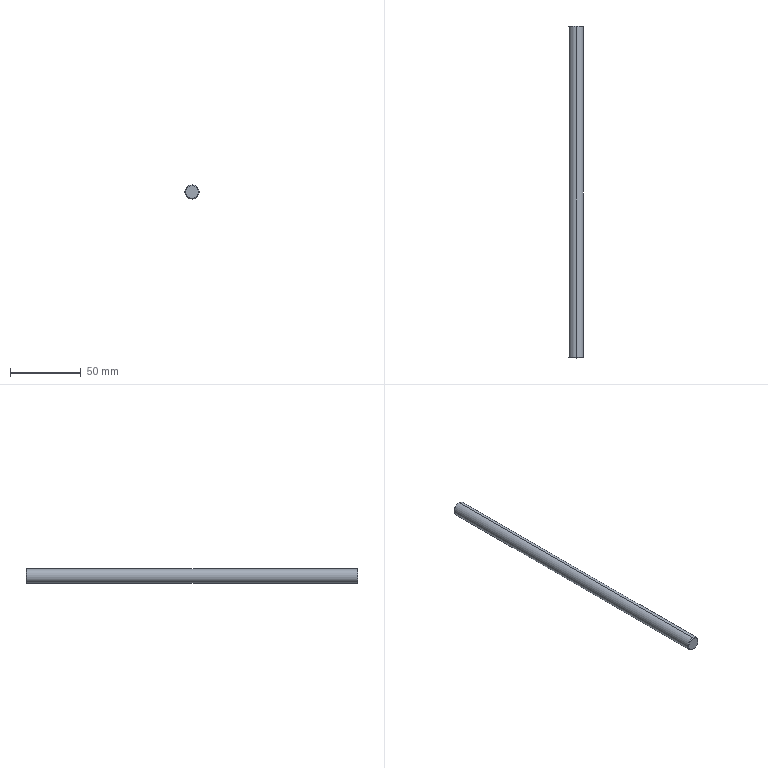Component | SolidWorks | STB-08-020-2 | 1 solid | 8 faces | box 10 x 235 x 10 mm | volume 18449 mm3 | cone 4 | cylinder 2 | plane 2 | commonest cylinder face diameters 10 x2
build123d program:
from build123d import *

# Parameters (mm, degrees)
SKETCH1_R           = 5
BOSS_EXTRUDE1_DEPTH = 117.5
CHAMFER1_SIZE       = 0.5


with BuildPart() as part:
    # Sketch1 → Boss-Extrude1 (new, symmetric)
    with BuildSketch(Plane(origin=(0, 0, 0), x_dir=(1, 0, 0), z_dir=(0, 1, 0))):
        with Locations(Location((0, 0, 0), (0, 0, 90))):
            Circle(SKETCH1_R)
    extrude(amount=BOSS_EXTRUDE1_DEPTH, both=True)

    # Chamfer1
    chamfer1_edges = [part.edges().sort_by_distance(p)[0] for p in [
        (0, -117.5, 5),
        (0, 117.5, 5),
    ]]
    chamfer(chamfer1_edges, length=CHAMFER1_SIZE)


solid = part.part

# Placed as in the assembly
solid = solid.moved(Location((-59.904, 349.499, -12), (0, 0, 0)))
STEP:
#1=COLOUR_RGB('',0.7922,0.8196,0.9333);
#2=FILL_AREA_STYLE_COLOUR('',#1);
#3=FILL_AREA_STYLE('',(#2));
#4=SURFACE_STYLE_FILL_AREA(#3);
#5=SURFACE_SIDE_STYLE('',(#4));
#6=SURFACE_STYLE_USAGE(.BOTH.,#5);
#7=PRESENTATION_STYLE_ASSIGNMENT((#6));
#8=CARTESIAN_POINT('',(-2.358,18.386,-0.2953));
#9=VERTEX_POINT('',#8);
#10=CARTESIAN_POINT('',(-2.358,18.386,-0.6496));
#11=VERTEX_POINT('',#10);
#12=CARTESIAN_POINT('',(-2.358,18.386,-0.4724));
#13=DIRECTION('',(0.,1.,0.));
#14=DIRECTION('',(0.,0.,1.));
#15=AXIS2_PLACEMENT_3D('',#12,#13,#14);
#16=CIRCLE('',#15,0.1772);
#17=EDGE_CURVE('',#9,#11,#16,.T.);
#18=ORIENTED_EDGE('',*,*,#17,.F.);
#19=CARTESIAN_POINT('',(-2.358,18.366,-0.2756));
#20=VERTEX_POINT('',#19);
#21=CARTESIAN_POINT('',(-2.358,18.386,-0.2953));
#22=DIRECTION('',(0.,-0.7071,0.7071));
#23=VECTOR('',#22,39.37);
#24=LINE('',#21,#23);
#25=EDGE_CURVE('',#9,#20,#24,.T.);
#26=ORIENTED_EDGE('',*,*,#25,.T.);
#27=CARTESIAN_POINT('',(-2.358,18.366,-0.6693));
#28=VERTEX_POINT('',#27);
#29=CARTESIAN_POINT('',(-2.358,18.366,-0.4724));
#30=DIRECTION('',(0.,-1.,0.));
#31=DIRECTION('',(0.,0.,1.));
#32=AXIS2_PLACEMENT_3D('',#29,#30,#31);
#33=CIRCLE('',#32,0.1969);
#34=EDGE_CURVE('',#28,#20,#33,.T.);
#35=ORIENTED_EDGE('',*,*,#34,.F.);
#36=CARTESIAN_POINT('',(-2.358,18.386,-0.6496));
#37=DIRECTION('',(0.,-0.7071,-0.7071));
#38=VECTOR('',#37,39.37);
#39=LINE('',#36,#38);
#40=EDGE_CURVE('',#11,#28,#39,.T.);
#41=ORIENTED_EDGE('',*,*,#40,.F.);
#42=EDGE_LOOP('',(#18,#26,#35,#41));
#43=FACE_OUTER_BOUND('',#42,.T.);
#44=CARTESIAN_POINT('',(-2.358,18.386,-0.4724));
#45=DIRECTION('',(0.,-1.,0.));
#46=DIRECTION('',(0.,0.,-1.));
#47=AXIS2_PLACEMENT_3D('',#44,#45,#46);
#48=CONICAL_SURFACE('',#47,0.1772,0.7854);
#49=ADVANCED_FACE('',(#43),#48,.T.);
#50=CARTESIAN_POINT('',(-2.358,9.134,-0.6496));
#51=VERTEX_POINT('',#50);
#52=CARTESIAN_POINT('',(-2.358,9.134,-0.2953));
#53=VERTEX_POINT('',#52);
#54=CARTESIAN_POINT('',(-2.358,9.134,-0.4724));
#55=DIRECTION('',(0.,-1.,0.));
#56=DIRECTION('',(0.,0.,1.));
#57=AXIS2_PLACEMENT_3D('',#54,#55,#56);
#58=CIRCLE('',#57,0.1772);
#59=EDGE_CURVE('',#51,#53,#58,.T.);
#60=ORIENTED_EDGE('',*,*,#59,.F.);
#61=CARTESIAN_POINT('',(-2.358,9.153,-0.6693));
#62=VERTEX_POINT('',#61);
#63=CARTESIAN_POINT('',(-2.358,9.153,-0.6693));
#64=DIRECTION('',(0.,0.7071,-0.7071));
#65=VECTOR('',#64,39.37);
#66=LINE('',#63,#65);
#67=EDGE_CURVE('',#51,#62,#66,.T.);
#68=ORIENTED_EDGE('',*,*,#67,.T.);
#69=CARTESIAN_POINT('',(-2.358,9.153,-0.2756));
#70=VERTEX_POINT('',#69);
#71=CARTESIAN_POINT('',(-2.358,9.153,-0.4724));
#72=DIRECTION('',(0.,1.,0.));
#73=DIRECTION('',(0.,0.,1.));
#74=AXIS2_PLACEMENT_3D('',#71,#72,#73);
#75=CIRCLE('',#74,0.1969);
#76=EDGE_CURVE('',#70,#62,#75,.T.);
#77=ORIENTED_EDGE('',*,*,#76,.F.);
#78=CARTESIAN_POINT('',(-2.358,9.153,-0.2756));
#79=DIRECTION('',(0.,0.7071,0.7071));
#80=VECTOR('',#79,39.37);
#81=LINE('',#78,#80);
#82=EDGE_CURVE('',#53,#70,#81,.T.);
#83=ORIENTED_EDGE('',*,*,#82,.F.);
#84=EDGE_LOOP('',(#60,#68,#77,#83));
#85=FACE_OUTER_BOUND('',#84,.T.);
#86=CARTESIAN_POINT('',(-2.358,9.153,-0.4724));
#87=DIRECTION('',(0.,1.,0.));
#88=DIRECTION('',(0.,0.,1.));
#89=AXIS2_PLACEMENT_3D('',#86,#87,#88);
#90=CONICAL_SURFACE('',#89,0.1969,0.7854);
#91=ADVANCED_FACE('',(#85),#90,.T.);
#92=ORIENTED_EDGE('',*,*,#34,.T.);
#93=CARTESIAN_POINT('',(-2.358,18.386,-0.2756));
#94=DIRECTION('',(0.,-1.,0.));
#95=VECTOR('',#94,39.37);
#96=LINE('',#93,#95);
#97=EDGE_CURVE('',#20,#70,#96,.T.);
#98=ORIENTED_EDGE('',*,*,#97,.T.);
#99=ORIENTED_EDGE('',*,*,#76,.T.);
#100=CARTESIAN_POINT('',(-2.358,18.386,-0.6693));
#101=DIRECTION('',(0.,-1.,0.));
#102=VECTOR('',#101,39.37);
#103=LINE('',#100,#102);
#104=EDGE_CURVE('',#28,#62,#103,.T.);
#105=ORIENTED_EDGE('',*,*,#104,.F.);
#106=EDGE_LOOP('',(#92,#98,#99,#105));
#107=FACE_OUTER_BOUND('',#106,.T.);
#108=CARTESIAN_POINT('',(-2.358,18.386,-0.4724));
#109=DIRECTION('',(0.,-1.,0.));
#110=DIRECTION('',(0.,0.,-1.));
#111=AXIS2_PLACEMENT_3D('',#108,#109,#110);
#112=CYLINDRICAL_SURFACE('',#111,0.1969);
#113=ADVANCED_FACE('',(#107),#112,.T.);
#114=ORIENTED_EDGE('',*,*,#97,.F.);
#115=CARTESIAN_POINT('',(-2.358,18.366,-0.4724));
#116=DIRECTION('',(0.,-1.,0.));
#117=DIRECTION('',(0.,0.,1.));
#118=AXIS2_PLACEMENT_3D('',#115,#116,#117);
#119=CIRCLE('',#118,0.1969);
#120=EDGE_CURVE('',#20,#28,#119,.T.);
#121=ORIENTED_EDGE('',*,*,#120,.T.);
#122=ORIENTED_EDGE('',*,*,#104,.T.);
#123=CARTESIAN_POINT('',(-2.358,9.153,-0.4724));
#124=DIRECTION('',(0.,1.,0.));
#125=DIRECTION('',(0.,0.,1.));
#126=AXIS2_PLACEMENT_3D('',#123,#124,#125);
#127=CIRCLE('',#126,0.1969);
#128=EDGE_CURVE('',#62,#70,#127,.T.);
#129=ORIENTED_EDGE('',*,*,#128,.T.);
#130=EDGE_LOOP('',(#114,#121,#122,#129));
#131=FACE_OUTER_BOUND('',#130,.T.);
#132=CARTESIAN_POINT('',(-2.358,18.386,-0.4724));
#133=DIRECTION('',(0.,-1.,0.));
#134=DIRECTION('',(0.,0.,-1.));
#135=AXIS2_PLACEMENT_3D('',#132,#133,#134);
#136=CYLINDRICAL_SURFACE('',#135,0.1969);
#137=ADVANCED_FACE('',(#131),#136,.T.);
#138=CARTESIAN_POINT('',(-2.358,18.386,-0.4724));
#139=DIRECTION('',(0.,1.,0.));
#140=DIRECTION('',(0.,0.,1.));
#141=AXIS2_PLACEMENT_3D('',#138,#139,#140);
#142=CIRCLE('',#141,0.1772);
#143=EDGE_CURVE('',#11,#9,#142,.T.);
#144=ORIENTED_EDGE('',*,*,#143,.T.);
#145=ORIENTED_EDGE('',*,*,#17,.T.);
#146=EDGE_LOOP('',(#144,#145));
#147=FACE_OUTER_BOUND('',#146,.T.);
#148=CARTESIAN_POINT('',(-2.358,18.386,-0.4724));
#149=DIRECTION('',(0.,1.,0.));
#150=DIRECTION('',(0.,0.,1.));
#151=AXIS2_PLACEMENT_3D('',#148,#149,#150);
#152=PLANE('',#151);
#153=ADVANCED_FACE('',(#147),#152,.T.);
#154=CARTESIAN_POINT('',(-2.358,9.134,-0.4724));
#155=DIRECTION('',(0.,-1.,0.));
#156=DIRECTION('',(0.,0.,1.));
#157=AXIS2_PLACEMENT_3D('',#154,#155,#156);
#158=CIRCLE('',#157,0.1772);
#159=EDGE_CURVE('',#53,#51,#158,.T.);
#160=ORIENTED_EDGE('',*,*,#159,.T.);
#161=ORIENTED_EDGE('',*,*,#59,.T.);
#162=EDGE_LOOP('',(#160,#161));
#163=FACE_OUTER_BOUND('',#162,.T.);
#164=CARTESIAN_POINT('',(-2.358,9.134,-0.4724));
#165=DIRECTION('',(0.,1.,0.));
#166=DIRECTION('',(0.,0.,1.));
#167=AXIS2_PLACEMENT_3D('',#164,#165,#166);
#168=PLANE('',#167);
#169=ADVANCED_FACE('',(#163),#168,.F.);
#170=ORIENTED_EDGE('',*,*,#67,.F.);
#171=ORIENTED_EDGE('',*,*,#159,.F.);
#172=ORIENTED_EDGE('',*,*,#82,.T.);
#173=ORIENTED_EDGE('',*,*,#128,.F.);
#174=EDGE_LOOP('',(#170,#171,#172,#173));
#175=FACE_OUTER_BOUND('',#174,.T.);
#176=CARTESIAN_POINT('',(-2.358,9.153,-0.4724));
#177=DIRECTION('',(0.,1.,0.));
#178=DIRECTION('',(0.,0.,1.));
#179=AXIS2_PLACEMENT_3D('',#176,#177,#178);
#180=CONICAL_SURFACE('',#179,0.1969,0.7854);
#181=ADVANCED_FACE('',(#175),#180,.T.);
#182=ORIENTED_EDGE('',*,*,#25,.F.);
#183=ORIENTED_EDGE('',*,*,#143,.F.);
#184=ORIENTED_EDGE('',*,*,#40,.T.);
#185=ORIENTED_EDGE('',*,*,#120,.F.);
#186=EDGE_LOOP('',(#182,#183,#184,#185));
#187=FACE_OUTER_BOUND('',#186,.T.);
#188=CARTESIAN_POINT('',(-2.358,18.386,-0.4724));
#189=DIRECTION('',(0.,-1.,0.));
#190=DIRECTION('',(0.,0.,-1.));
#191=AXIS2_PLACEMENT_3D('',#188,#189,#190);
#192=CONICAL_SURFACE('',#191,0.1772,0.7854);
#193=ADVANCED_FACE('',(#187),#192,.T.);
#194=CLOSED_SHELL('',(#49,#91,#113,#137,#153,#169,#181,#193));
#195=MANIFOLD_SOLID_BREP('',#194);
#196=STYLED_ITEM('',(#7),#195);
#197=(LENGTH_UNIT()NAMED_UNIT(*)SI_UNIT($,.METRE.));
#198=LENGTH_MEASURE_WITH_UNIT(LENGTH_MEASURE(0.0254),#197);
#199=DIMENSIONAL_EXPONENTS(1.,0.,0.,0.,0.,0.,0.);
#200=(CONVERSION_BASED_UNIT('',#198)LENGTH_UNIT()NAMED_UNIT(#199));
#201=UNCERTAINTY_MEASURE_WITH_UNIT(LENGTH_MEASURE(0.00001),#200,'','');
#202=(NAMED_UNIT(*)PLANE_ANGLE_UNIT()SI_UNIT($,.RADIAN.));
#203=(NAMED_UNIT(*)SI_UNIT($,.STERADIAN.)SOLID_ANGLE_UNIT());
#204=(GEOMETRIC_REPRESENTATION_CONTEXT(3)GLOBAL_UNCERTAINTY_ASSIGNED_CONTEXT((#201))GLOBAL_UNIT_ASSIGNED_CONTEXT((#200,#202,#203))REPRESENTATION_CONTEXT('',''));
#205=MECHANICAL_DESIGN_GEOMETRIC_PRESENTATION_REPRESENTATION('',(#196),#204);
#206=PRESENTATION_LAYER_ASSIGNMENT('','',(#196));
#207=CARTESIAN_POINT('',(0.,0.,0.));
#208=DIRECTION('',(0.,0.,1.));
#209=DIRECTION('',(1.,0.,0.));
#210=AXIS2_PLACEMENT_3D('',#207,#208,#209);
#211=(LENGTH_UNIT()NAMED_UNIT(*)SI_UNIT($,.METRE.));
#212=LENGTH_MEASURE_WITH_UNIT(LENGTH_MEASURE(0.0254),#211);
#213=DIMENSIONAL_EXPONENTS(1.,0.,0.,0.,0.,0.,0.);
#214=(CONVERSION_BASED_UNIT('',#212)LENGTH_UNIT()NAMED_UNIT(#213));
#215=UNCERTAINTY_MEASURE_WITH_UNIT(LENGTH_MEASURE(0.00001),#214,'','');
#216=(NAMED_UNIT(*)PLANE_ANGLE_UNIT()SI_UNIT($,.RADIAN.));
#217=(NAMED_UNIT(*)SI_UNIT($,.STERADIAN.)SOLID_ANGLE_UNIT());
#218=(GEOMETRIC_REPRESENTATION_CONTEXT(3)GLOBAL_UNCERTAINTY_ASSIGNED_CONTEXT((#215))GLOBAL_UNIT_ASSIGNED_CONTEXT((#214,#216,#217))REPRESENTATION_CONTEXT('',''));
#219=ADVANCED_BREP_SHAPE_REPRESENTATION('',(#195,#210),#218);